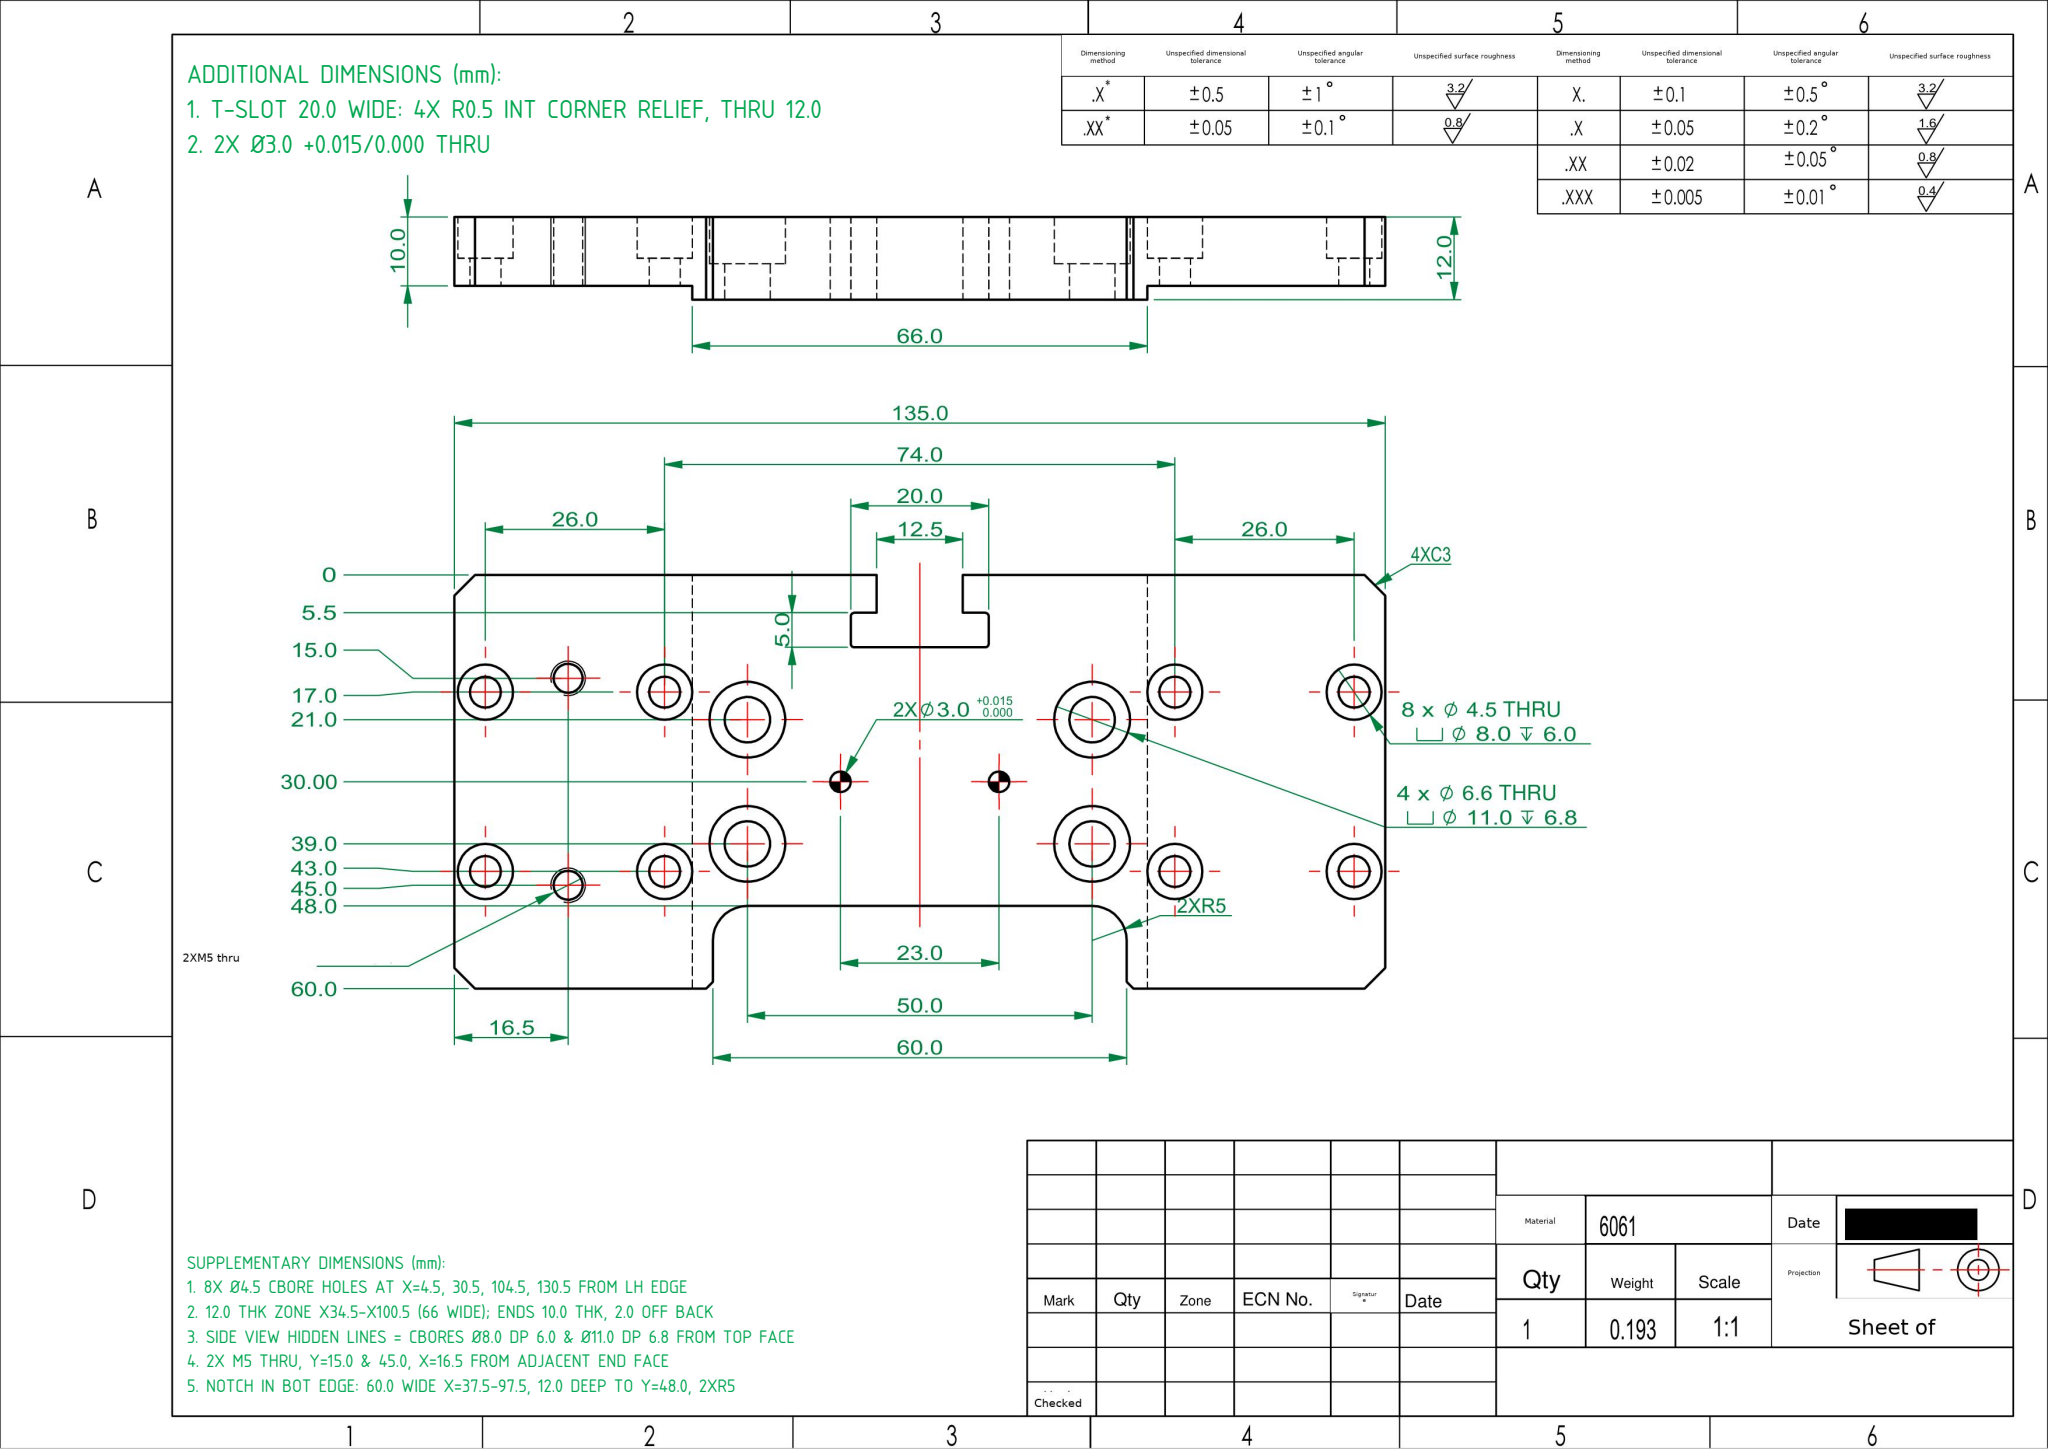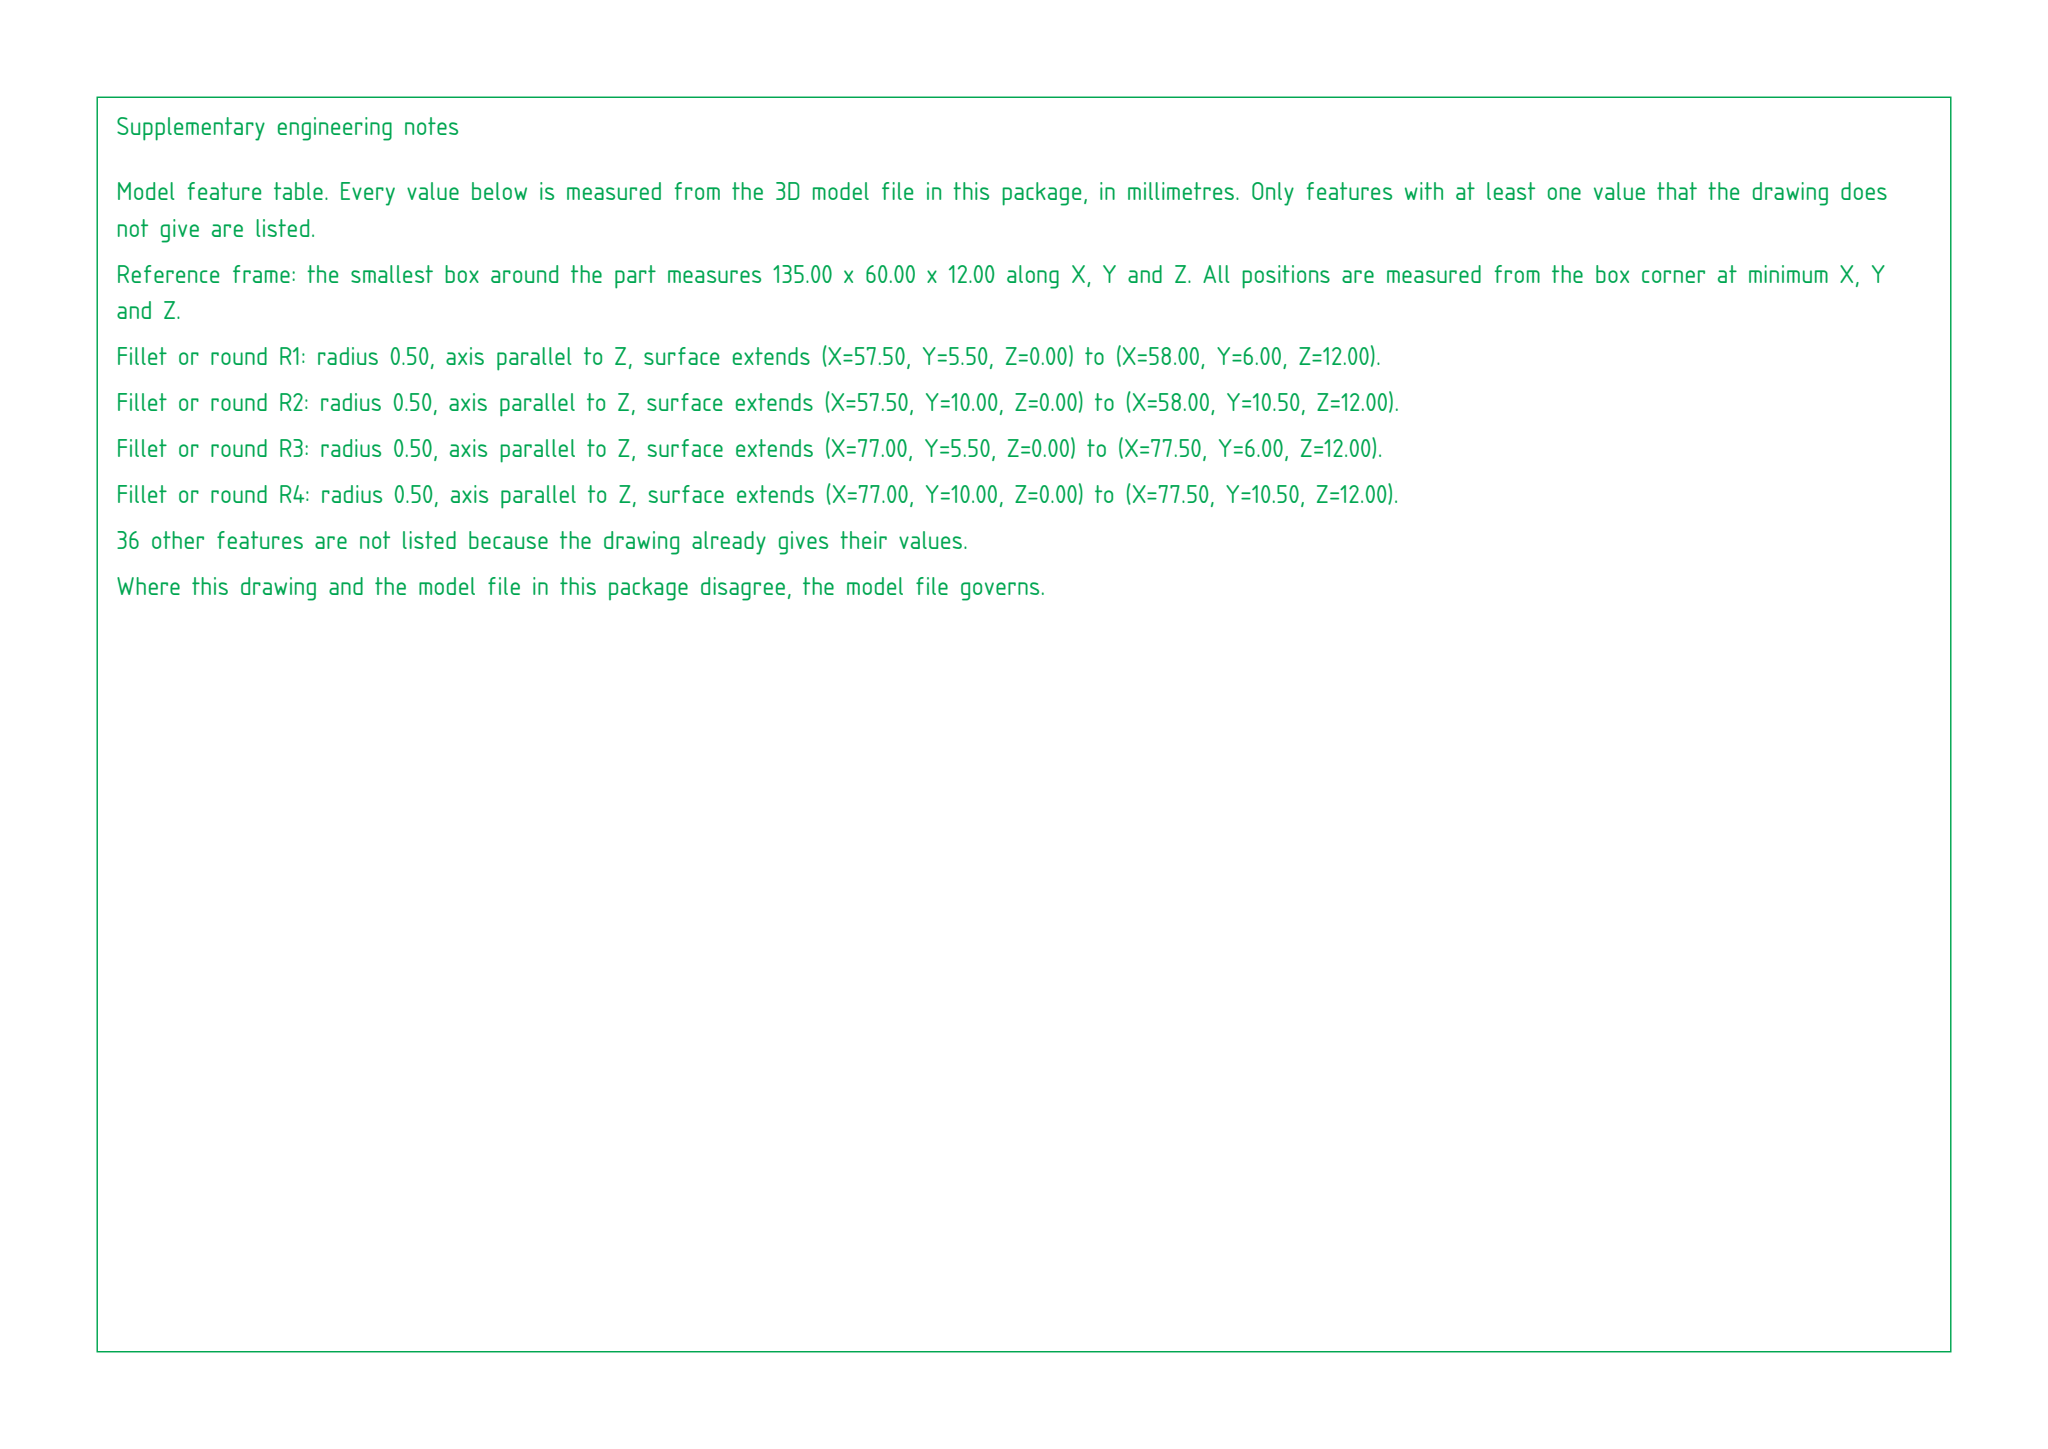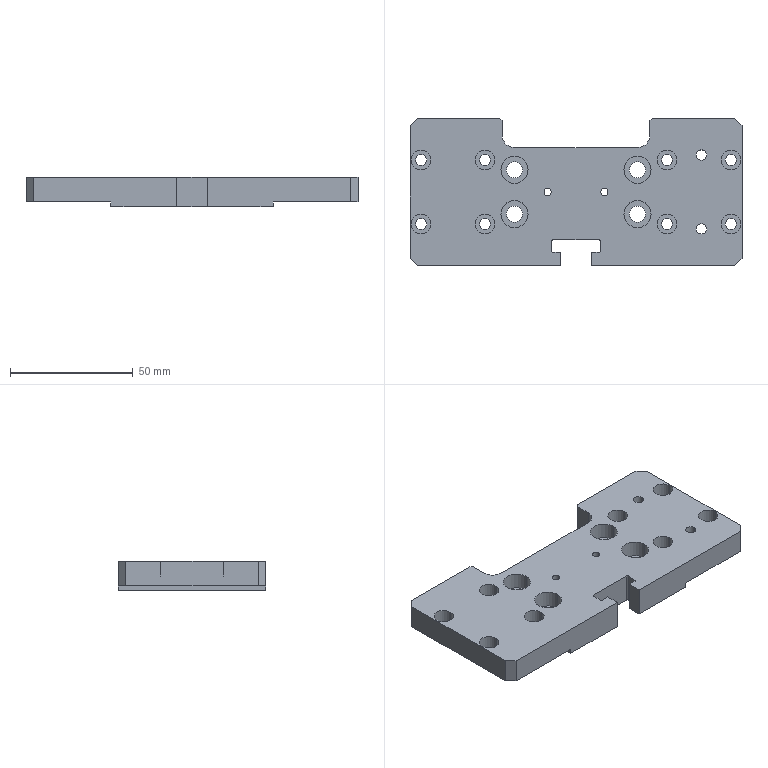Part | SolidWorks | mm | 1 solid | 102 faces | box 135 x 60 x 12 mm | volume 71529 mm3 | cylinder 62 | plane 40 | commonest cylinder face diameters 8 x16 4.5 x16 11 x8 6.6 x8 4.2 x4 3 x4 1 x4 10 x2
build123d program:
from build123d import *

# Parameters (mm, degrees)
SKETCH1_W                                         = 135
SKETCH1_H                                         = 60
BOSS_EXTRUDE1_DEPTH                               = 12
HOLE_SIZE_ACCORDING_TO_HEXAGON_SOCKET_D           = 4.5
HOLE_SIZE_ACCORDING_TO_HEXAGON_SOCKET_CBORE_D     = 8
HOLE_SIZE_ACCORDING_TO_HEXAGON_SOCKET_CBORE_DEPTH = 6
SKETCH6_OUTSIDE_W                                 = 166.644
SKETCH6_OUTSIDE_H                                 = 91.644
SKETCH6_OUTSIDE_W_2                               = 66
SKETCH6_OUTSIDE_H_2                               = 60
CUT_EXTRUDE3_DEPTH                                = 2
HOLE_SIZE_ACCORDING_TO_HEXAGON_SO_2_D             = 6.6
HOLE_SIZE_ACCORDING_TO_HEXAGON_SO_2_CBORE_D       = 11
HOLE_SIZE_ACCORDING_TO_HEXAGON_SO_2_CBORE_DEPTH   = 6.8
SKETCH12_W                                        = 12.5
SKETCH12_H                                        = 16
CUT_EXTRUDE4_DEPTH                                = 21
SKETCH13_W                                        = 20
SKETCH13_H                                        = 5
CUT_EXTRUDE5_DEPTH                                = 21
CHAMFER1_SIZE                                     = 3
FILLET1_R                                         = 0.5
SIZE_MM_DOWEL_PIN_HOLE_1_D                        = 3
SKETCH16_W                                        = 60
SKETCH16_H                                        = 24
CUT_EXTRUDE6_DEPTH                                = 46
FILLET2_R                                         = 5
M5_TAPPED_HOLE1_D                                 = 4.2
M5_TAPPED_HOLE1_DEPTH                             = 14
M5_TAPPED_HOLE1_TIP                               = 1.262
CHAMFER2_SIZE                                     = 1


with BuildPart() as part:
    # Sketch1 → Boss-Extrude1 (new body)
    with BuildSketch(Plane.XY):
        Rectangle(SKETCH1_W, SKETCH1_H)
    extrude(amount=BOSS_EXTRUDE1_DEPTH)

    # Hole Size _ according to_ Hexagon Socket (through all)
    with Locations(Plane(origin=(-63, 13, 12), x_dir=(1, 0, 0), z_dir=(0, 0, 1))):
        with Locations((0, 0), (26, 0), (26, -26), (0, -26), (100, 0), (126, 0), (126, -26), (100, -26)):
            CounterBoreHole(HOLE_SIZE_ACCORDING_TO_HEXAGON_SOCKET_D / 2, HOLE_SIZE_ACCORDING_TO_HEXAGON_SOCKET_CBORE_D / 2, HOLE_SIZE_ACCORDING_TO_HEXAGON_SOCKET_CBORE_DEPTH)

    # Sketch6 outside → Cut-Extrude3 (cut)
    with BuildSketch(Plane(origin=(0, 0, 0), x_dir=(-1, 0, 0), z_dir=(0, 0, -1))):
        Rectangle(SKETCH6_OUTSIDE_W, SKETCH6_OUTSIDE_H)
        Rectangle(SKETCH6_OUTSIDE_W_2, SKETCH6_OUTSIDE_H_2, mode=Mode.SUBTRACT)
    extrude(amount=-CUT_EXTRUDE3_DEPTH, mode=Mode.SUBTRACT)

    # Hole Size _ according to_ Hexagon So 2 (through all)
    with Locations(Plane(origin=(-25, 9, 12), x_dir=(1, 0, 0), z_dir=(0, 0, 1))):
        with Locations((0, 0), (0, -18), (50, -18), (50, 0)):
            CounterBoreHole(HOLE_SIZE_ACCORDING_TO_HEXAGON_SO_2_D / 2, HOLE_SIZE_ACCORDING_TO_HEXAGON_SO_2_CBORE_D / 2, HOLE_SIZE_ACCORDING_TO_HEXAGON_SO_2_CBORE_DEPTH)

    # Sketch12 → Cut-Extrude4 (cut)
    with BuildSketch(Plane.XY.offset(12)):
        with Locations((0, -30)):
            Rectangle(SKETCH12_W, SKETCH12_H)
    extrude(amount=-CUT_EXTRUDE4_DEPTH, mode=Mode.SUBTRACT)

    # Sketch13 → Cut-Extrude5 (cut)
    with BuildSketch(Plane.XY.offset(12)):
        with Locations((0, -22)):
            Rectangle(SKETCH13_W, SKETCH13_H)
    extrude(amount=-CUT_EXTRUDE5_DEPTH, mode=Mode.SUBTRACT)

    # Chamfer1
    chamfer1_edges = [part.edges().sort_by_distance(p)[0] for p in [
        (67.5, -30, 7),
        (-67.5, -30, 7),
        (-67.5, 30, 7),
        (67.5, 30, 7),
    ]]
    chamfer(chamfer1_edges, length=CHAMFER1_SIZE)

    # Fillet1
    fillet1_edges = [part.edges().sort_by_distance(p)[0] for p in [
        (10, -19.5, 6),
        (-10, -24.5, 6),
        (-10, -19.5, 6),
        (10, -24.5, 6),
    ]]
    fillet(fillet1_edges, radius=FILLET1_R)

    # Size mm Dowel Pin Hole 1 (through all)
    with Locations(Plane(origin=(-11.5, 0, 12), x_dir=(1, 0, 0), z_dir=(0, 0, 1))):
        with Locations((0, 0), (23, 0)):
            Hole(SIZE_MM_DOWEL_PIN_HOLE_1_D / 2)

    # Sketch16 → Cut-Extrude6 (cut)
    with BuildSketch(Plane.XY.offset(12)):
        with Locations((0, 30)):
            Rectangle(SKETCH16_W, SKETCH16_H)
    extrude(amount=-CUT_EXTRUDE6_DEPTH, mode=Mode.SUBTRACT)

    # Fillet2
    fillet2_edges = [part.edges().sort_by_distance(p)[0] for p in [
        (30, 18, 6),
        (-30, 18, 6),
    ]]
    fillet(fillet2_edges, radius=FILLET2_R)

    # M5 Tapped Hole1
    with Locations(Plane(origin=(51, 15, 12), x_dir=(1, 0, 0), z_dir=(0, 0, 1))):
        with Locations((0, 0), (0, -30)):
            Hole(M5_TAPPED_HOLE1_D / 2, depth=M5_TAPPED_HOLE1_DEPTH)
            with Locations((0, 0, -(M5_TAPPED_HOLE1_DEPTH + M5_TAPPED_HOLE1_TIP / 2))):  # 118° drill point
                Cone(0, M5_TAPPED_HOLE1_D / 2, M5_TAPPED_HOLE1_TIP, mode=Mode.SUBTRACT)

    # Chamfer2
    chamfer2_edges = [part.edges().sort_by_distance(p)[0] for p in [
        (30, 30, 6),
        (-30, 30, 6),
    ]]
    chamfer(chamfer2_edges, length=CHAMFER2_SIZE)


solid = part.part